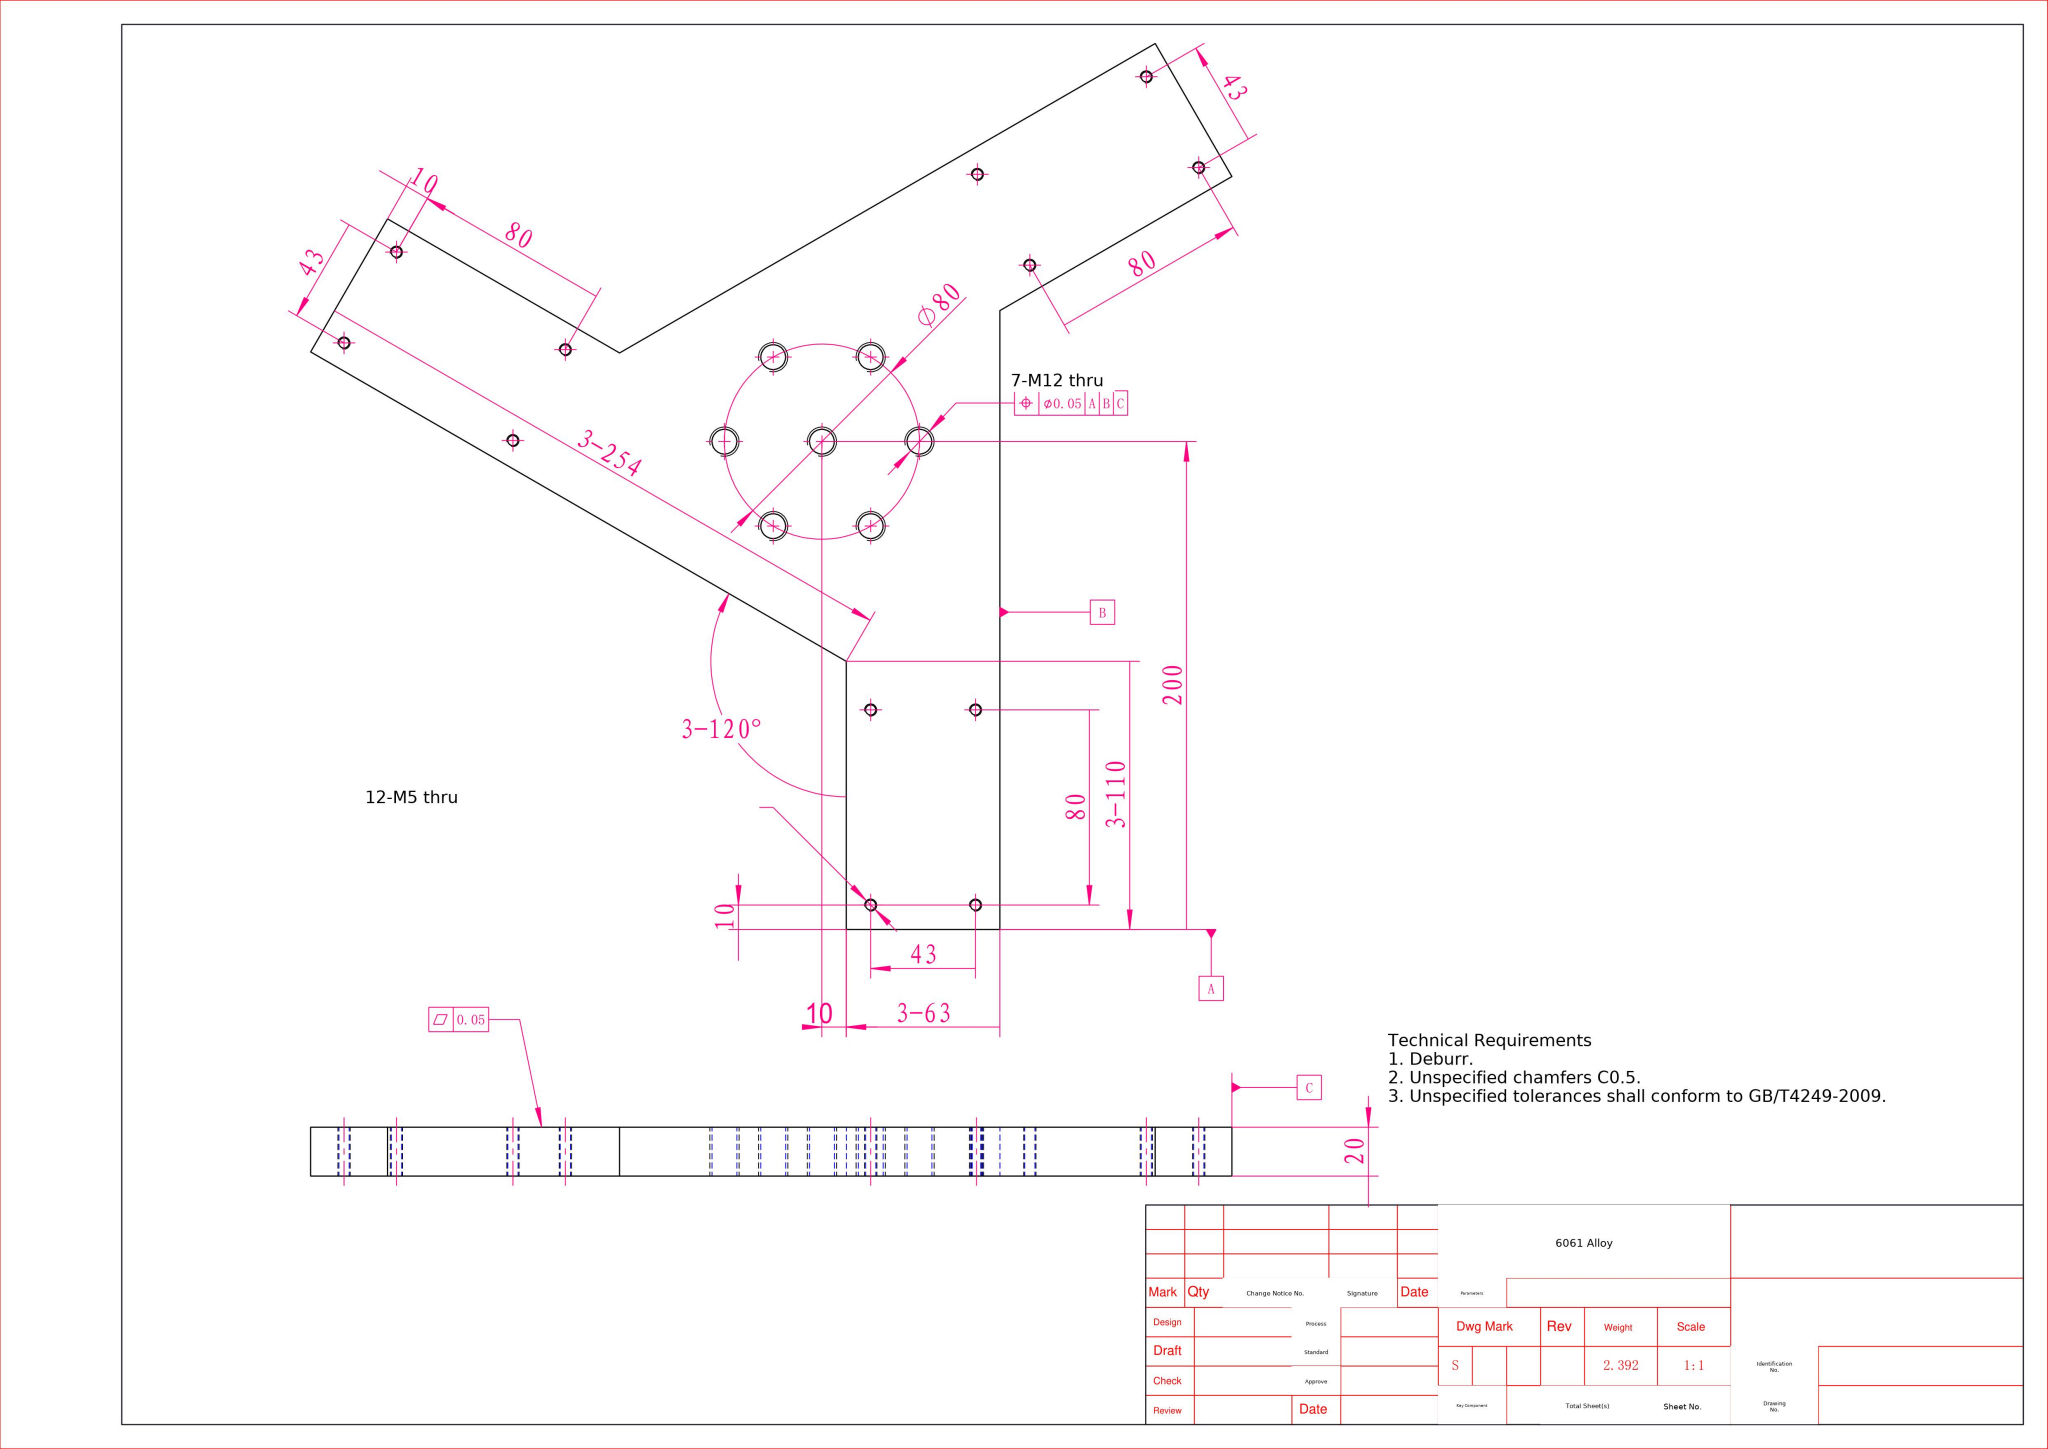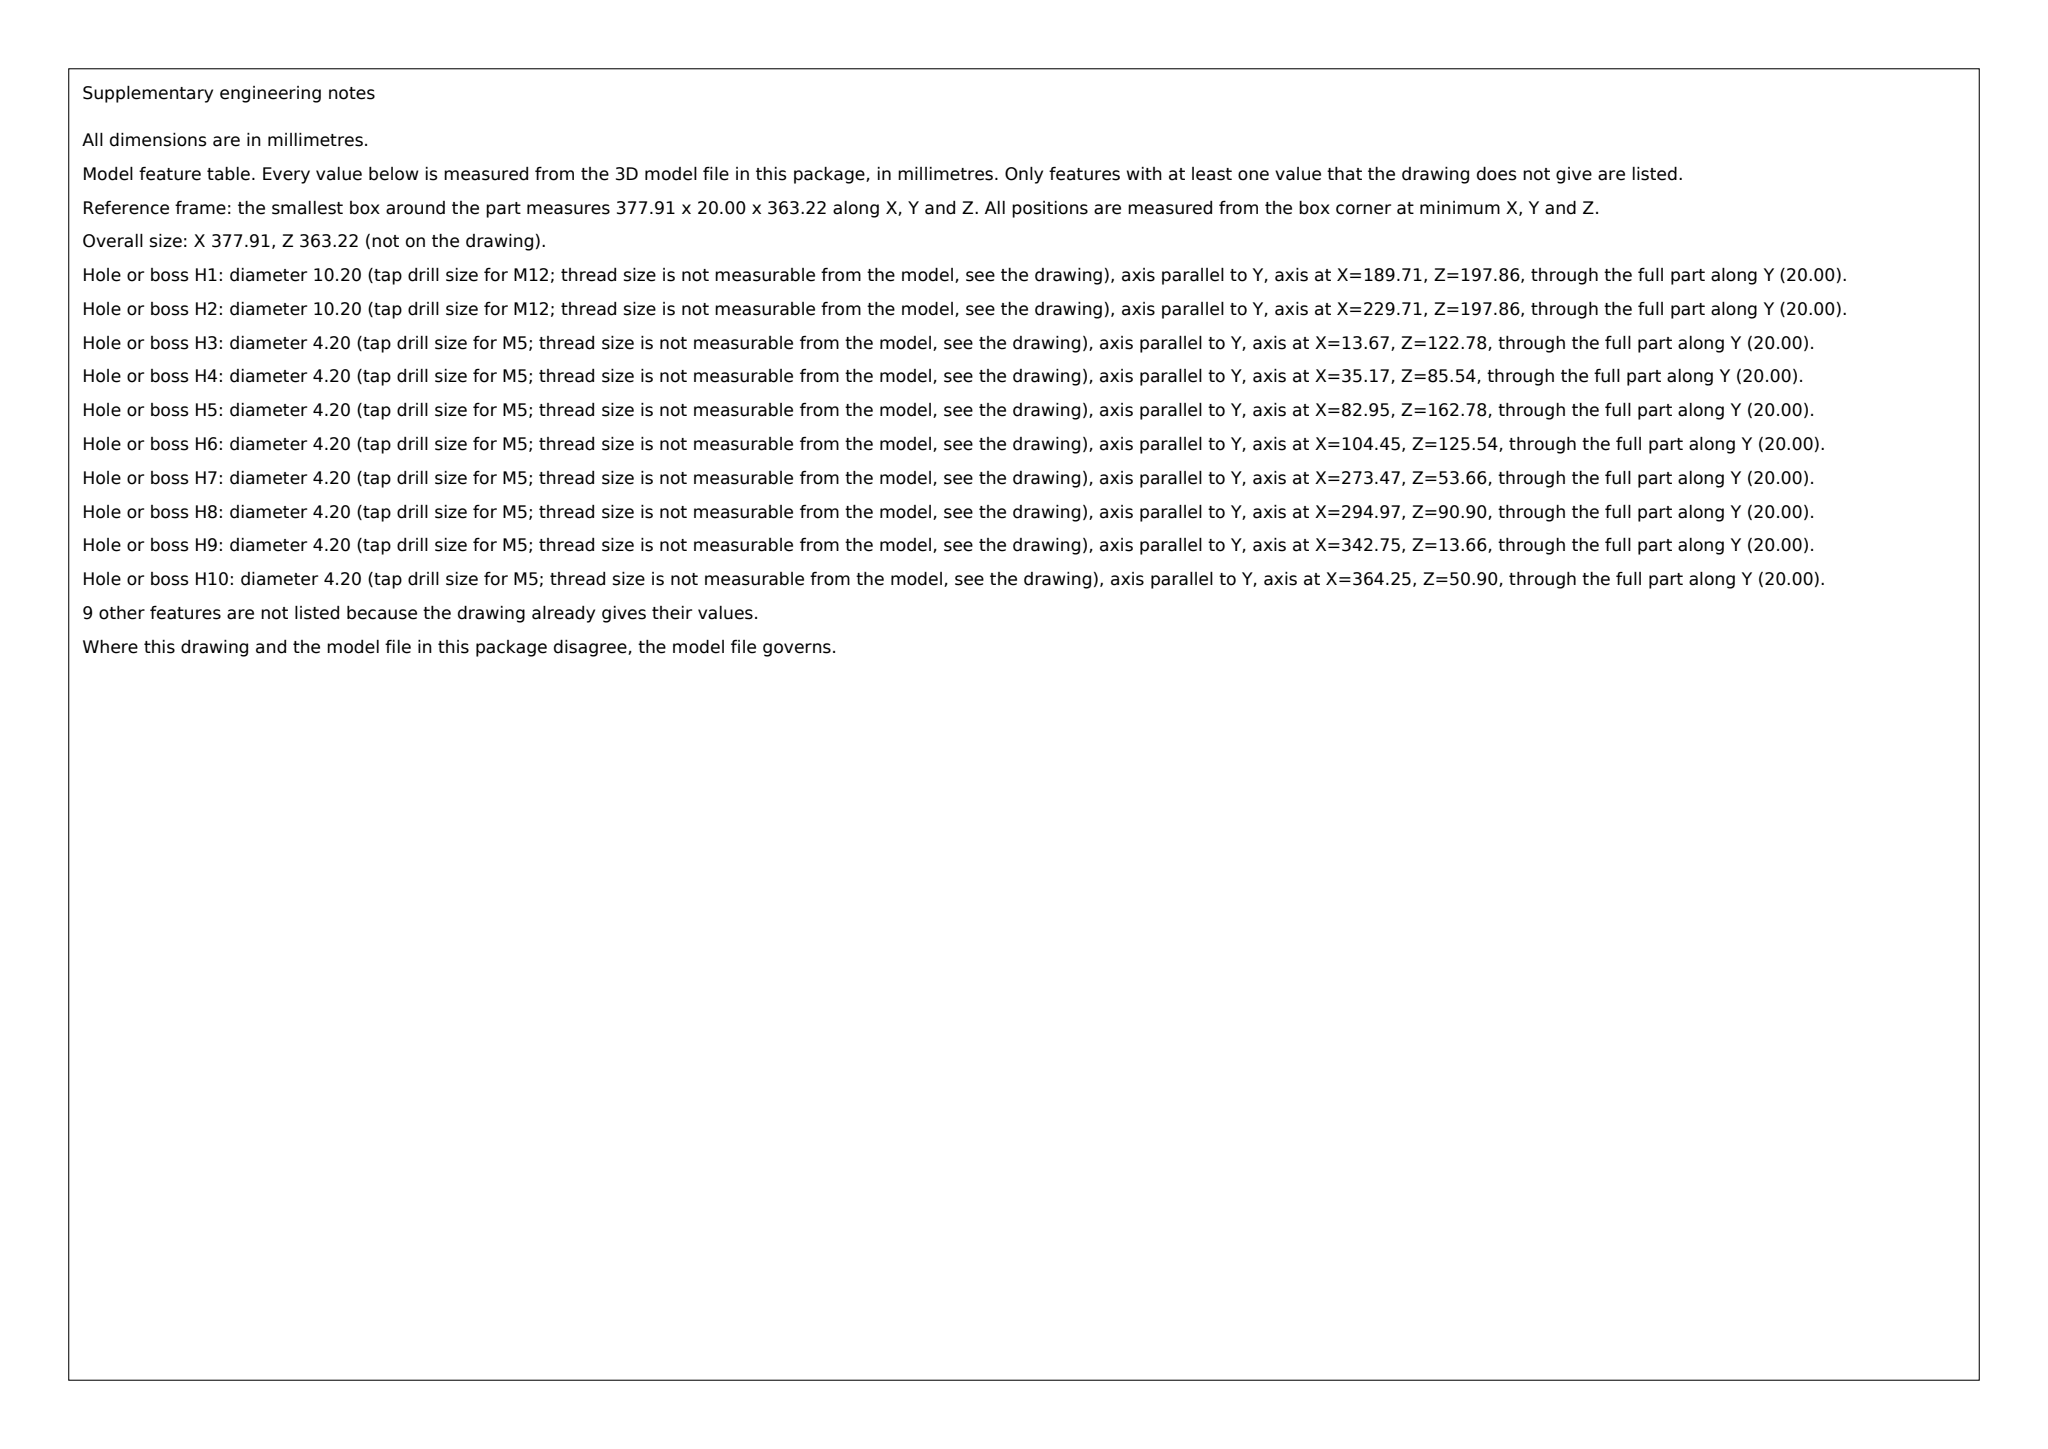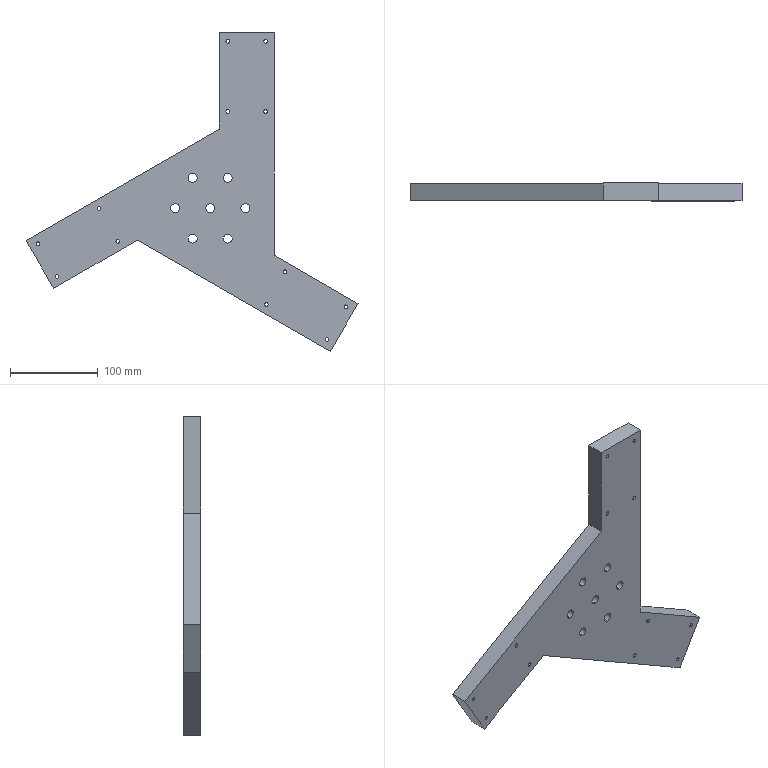Part | SolidWorks | mm | material 6061 Alloy | 1 solid | 49 faces | box 377.91 x 20 x 363.22 mm | volume 885844 mm3 | cylinder 38 | plane 11 | commonest cylinder face diameters 4.2 x24 10.2 x14